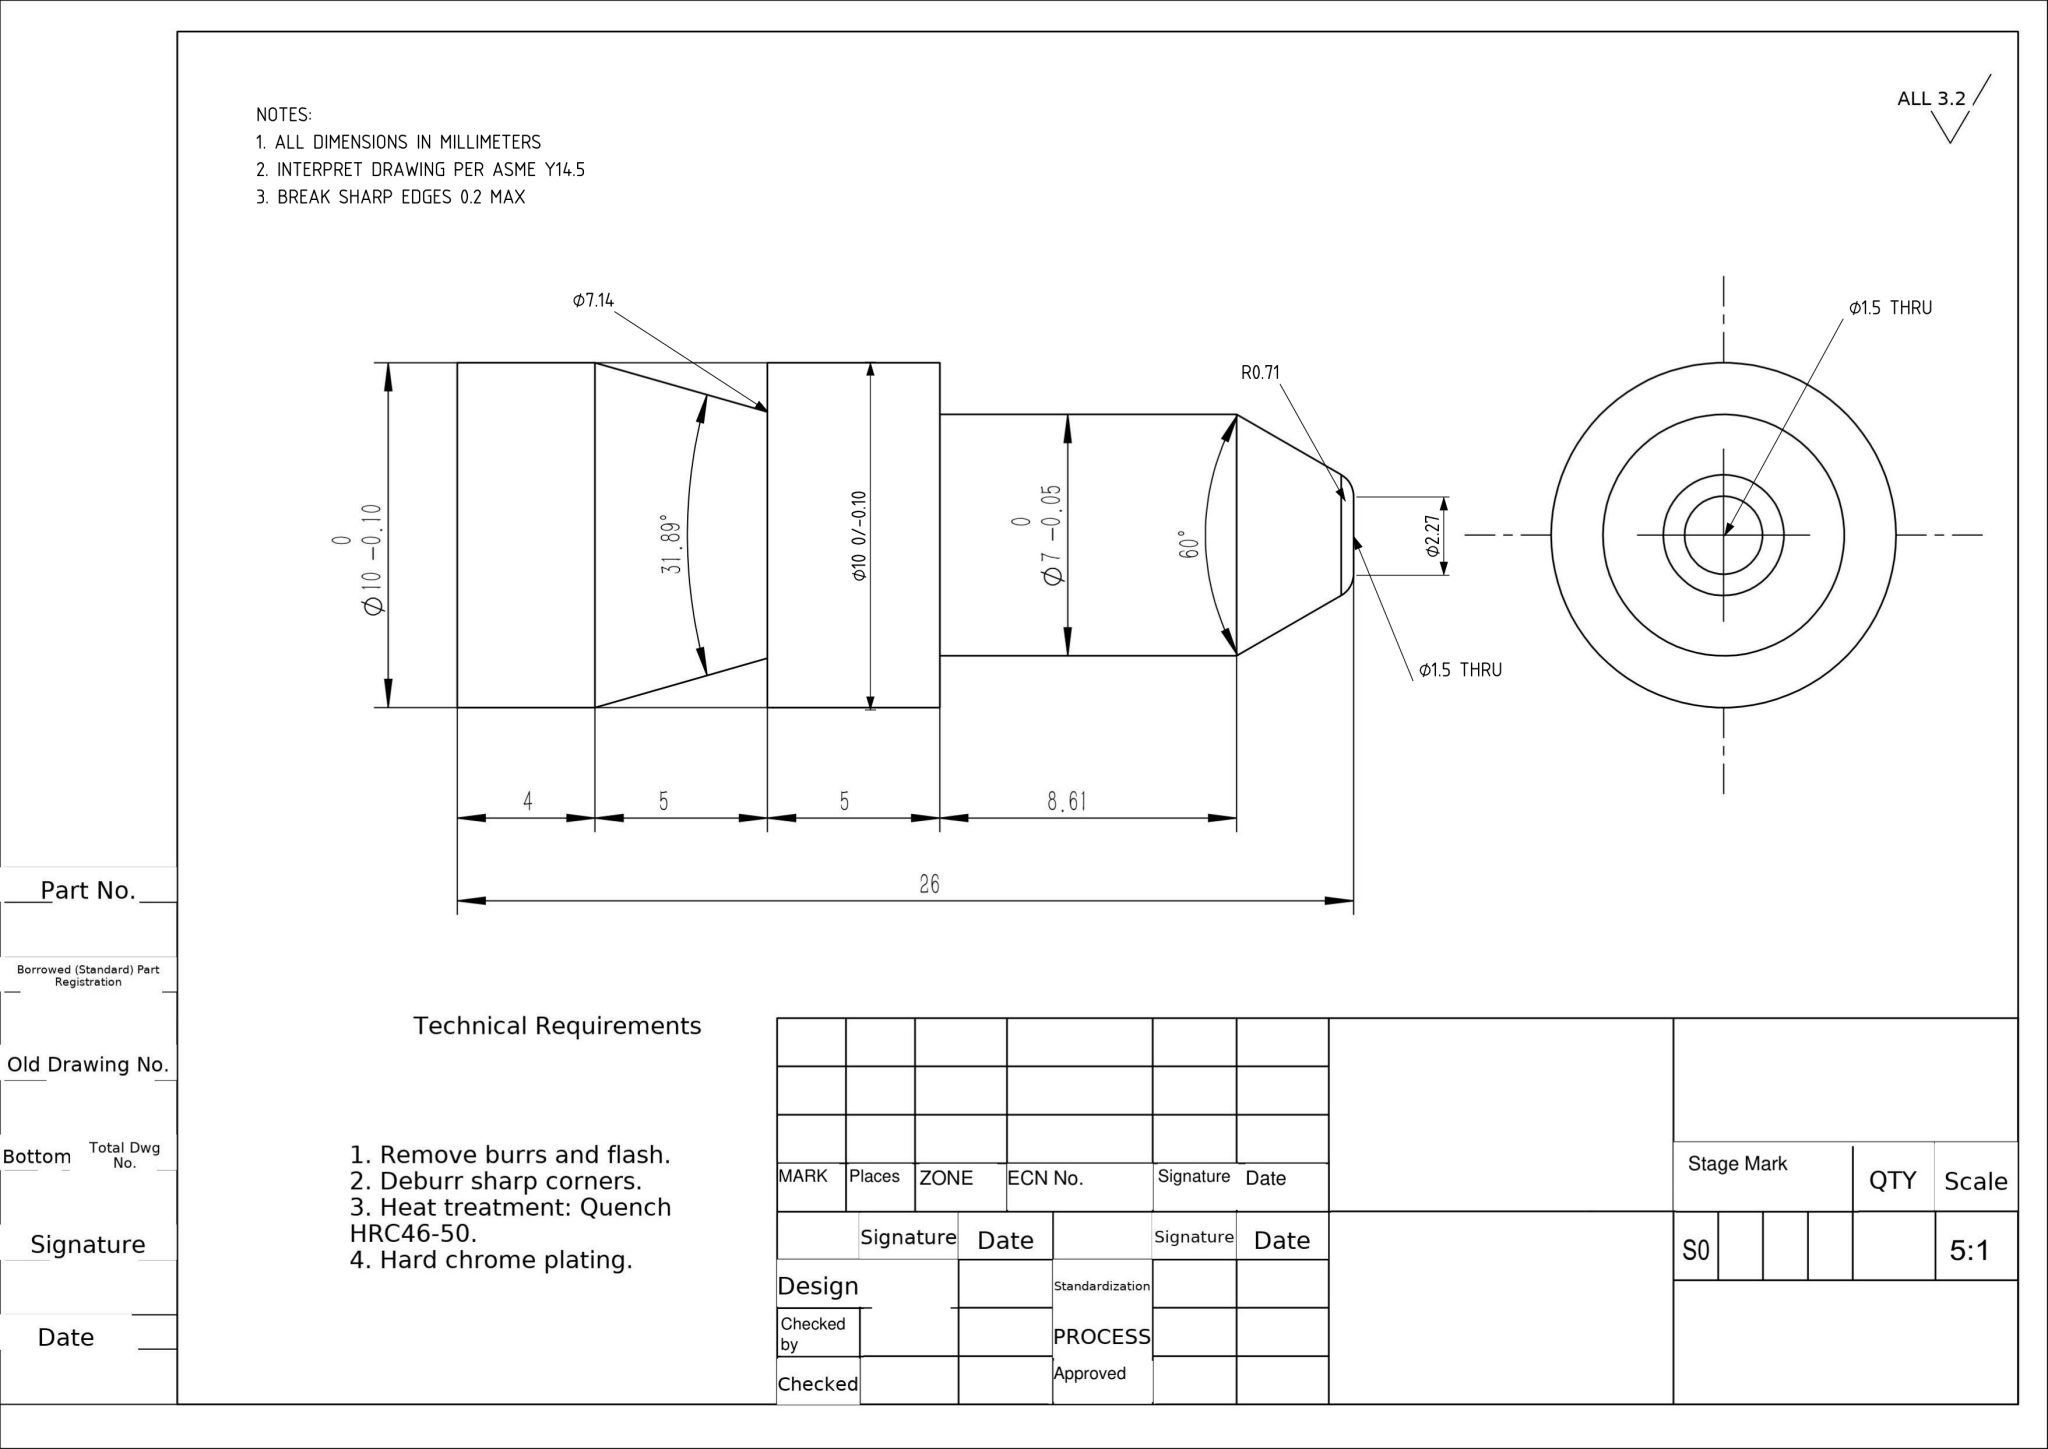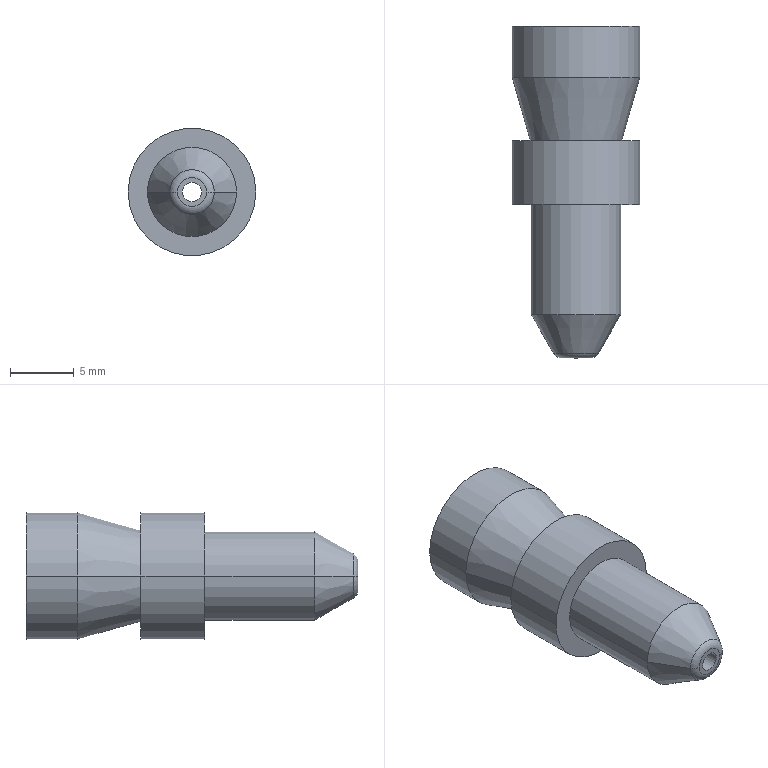Part | NX | mm | 1 solid | 18 faces | box 10 x 26 x 10 mm | volume 1354 mm3 | cylinder 8 | cone 4 | plane 4 | torus 2 | commonest cylinder face diameters 10 x4 1.5 x2 7 x2
STEP:
#1=COLOUR_RGB('',0.7922,0.8196,0.9333);
#2=FILL_AREA_STYLE_COLOUR('',#1);
#3=FILL_AREA_STYLE('',(#2));
#4=SURFACE_STYLE_FILL_AREA(#3);
#5=SURFACE_SIDE_STYLE('',(#4));
#6=SURFACE_STYLE_USAGE(.BOTH.,#5);
#7=PRESENTATION_STYLE_ASSIGNMENT((#6));
#8=CARTESIAN_POINT('',(1.464,7.397,0.));
#9=VERTEX_POINT('',#8);
#10=CARTESIAN_POINT('',(-0.03571,7.397,0.));
#11=VERTEX_POINT('',#10);
#12=CARTESIAN_POINT('',(0.7143,7.397,0.));
#13=DIRECTION('',(-0.,1.,0.));
#14=DIRECTION('',(-1.,0.,0.));
#15=AXIS2_PLACEMENT_3D('',#12,#13,#14);
#16=CIRCLE('',#15,0.75);
#17=EDGE_CURVE('',#9,#11,#16,.T.);
#18=ORIENTED_EDGE('',*,*,#17,.F.);
#19=CARTESIAN_POINT('',(1.464,33.397,0.));
#20=VERTEX_POINT('',#19);
#21=CARTESIAN_POINT('',(1.464,7.397,0.));
#22=DIRECTION('',(-0.,1.,0.));
#23=VECTOR('',#22,1000.);
#24=LINE('',#21,#23);
#25=EDGE_CURVE('',#9,#20,#24,.T.);
#26=ORIENTED_EDGE('',*,*,#25,.T.);
#27=CARTESIAN_POINT('',(-0.03571,33.397,0.));
#28=VERTEX_POINT('',#27);
#29=CARTESIAN_POINT('',(0.7143,33.397,0.));
#30=DIRECTION('',(-0.,1.,0.));
#31=DIRECTION('',(-1.,0.,0.));
#32=AXIS2_PLACEMENT_3D('',#29,#30,#31);
#33=CIRCLE('',#32,0.75);
#34=EDGE_CURVE('',#20,#28,#33,.T.);
#35=ORIENTED_EDGE('',*,*,#34,.T.);
#36=CARTESIAN_POINT('',(-0.03571,7.397,0.));
#37=DIRECTION('',(-0.,1.,0.));
#38=VECTOR('',#37,1000.);
#39=LINE('',#36,#38);
#40=EDGE_CURVE('',#11,#28,#39,.T.);
#41=ORIENTED_EDGE('',*,*,#40,.F.);
#42=EDGE_LOOP('',(#18,#26,#35,#41));
#43=FACE_OUTER_BOUND('',#42,.T.);
#44=CARTESIAN_POINT('',(0.7143,7.397,0.));
#45=DIRECTION('',(-0.,1.,0.));
#46=DIRECTION('',(-1.,0.,0.));
#47=AXIS2_PLACEMENT_3D('',#44,#45,#46);
#48=CYLINDRICAL_SURFACE('',#47,0.75);
#49=ADVANCED_FACE('',(#43),#48,.F.);
#50=CARTESIAN_POINT('',(2.464,7.755,0.));
#51=VERTEX_POINT('',#50);
#52=CARTESIAN_POINT('',(4.214,10.786,0.));
#53=VERTEX_POINT('',#52);
#54=CARTESIAN_POINT('',(4.214,10.786,0.));
#55=DIRECTION('',(0.5,0.866,0.));
#56=VECTOR('',#55,1000.);
#57=LINE('',#54,#56);
#58=EDGE_CURVE('',#51,#53,#57,.T.);
#59=ORIENTED_EDGE('',*,*,#58,.F.);
#60=CARTESIAN_POINT('',(-1.036,7.755,0.));
#61=VERTEX_POINT('',#60);
#62=CARTESIAN_POINT('',(0.7143,7.755,0.));
#63=DIRECTION('',(0.,1.,0.));
#64=DIRECTION('',(-1.,0.,0.));
#65=AXIS2_PLACEMENT_3D('',#62,#63,#64);
#66=CIRCLE('',#65,1.75);
#67=EDGE_CURVE('',#51,#61,#66,.T.);
#68=ORIENTED_EDGE('',*,*,#67,.T.);
#69=CARTESIAN_POINT('',(-2.786,10.786,0.));
#70=VERTEX_POINT('',#69);
#71=CARTESIAN_POINT('',(-2.786,10.786,0.));
#72=DIRECTION('',(-0.5,0.866,0.));
#73=VECTOR('',#72,1000.);
#74=LINE('',#71,#73);
#75=EDGE_CURVE('',#61,#70,#74,.T.);
#76=ORIENTED_EDGE('',*,*,#75,.T.);
#77=CARTESIAN_POINT('',(0.7143,10.786,0.));
#78=DIRECTION('',(0.,1.,0.));
#79=DIRECTION('',(-1.,0.,0.));
#80=AXIS2_PLACEMENT_3D('',#77,#78,#79);
#81=CIRCLE('',#80,3.5);
#82=EDGE_CURVE('',#53,#70,#81,.T.);
#83=ORIENTED_EDGE('',*,*,#82,.F.);
#84=EDGE_LOOP('',(#59,#68,#76,#83));
#85=FACE_OUTER_BOUND('',#84,.T.);
#86=CARTESIAN_POINT('',(0.7143,10.786,0.));
#87=DIRECTION('',(0.,1.,0.));
#88=DIRECTION('',(-1.,0.,0.));
#89=AXIS2_PLACEMENT_3D('',#86,#87,#88);
#90=CONICAL_SURFACE('',#89,3.5,0.5236);
#91=ADVANCED_FACE('',(#85),#90,.T.);
#92=CARTESIAN_POINT('',(4.214,19.397,0.));
#93=VERTEX_POINT('',#92);
#94=CARTESIAN_POINT('',(4.214,7.397,0.));
#95=DIRECTION('',(-0.,1.,0.));
#96=VECTOR('',#95,1000.);
#97=LINE('',#94,#96);
#98=EDGE_CURVE('',#53,#93,#97,.T.);
#99=ORIENTED_EDGE('',*,*,#98,.F.);
#100=ORIENTED_EDGE('',*,*,#82,.T.);
#101=CARTESIAN_POINT('',(-2.786,19.397,0.));
#102=VERTEX_POINT('',#101);
#103=CARTESIAN_POINT('',(-2.786,7.397,0.));
#104=DIRECTION('',(-0.,1.,0.));
#105=VECTOR('',#104,1000.);
#106=LINE('',#103,#105);
#107=EDGE_CURVE('',#70,#102,#106,.T.);
#108=ORIENTED_EDGE('',*,*,#107,.T.);
#109=CARTESIAN_POINT('',(0.7143,19.397,0.));
#110=DIRECTION('',(0.,1.,0.));
#111=DIRECTION('',(-1.,0.,0.));
#112=AXIS2_PLACEMENT_3D('',#109,#110,#111);
#113=CIRCLE('',#112,3.5);
#114=EDGE_CURVE('',#93,#102,#113,.T.);
#115=ORIENTED_EDGE('',*,*,#114,.F.);
#116=EDGE_LOOP('',(#99,#100,#108,#115));
#117=FACE_OUTER_BOUND('',#116,.T.);
#118=CARTESIAN_POINT('',(0.7143,7.397,0.));
#119=DIRECTION('',(0.,1.,0.));
#120=DIRECTION('',(-1.,0.,0.));
#121=AXIS2_PLACEMENT_3D('',#118,#119,#120);
#122=CYLINDRICAL_SURFACE('',#121,3.5);
#123=ADVANCED_FACE('',(#117),#122,.T.);
#124=CARTESIAN_POINT('',(0.7143,19.397,0.));
#125=DIRECTION('',(0.,1.,0.));
#126=DIRECTION('',(-1.,0.,0.));
#127=AXIS2_PLACEMENT_3D('',#124,#125,#126);
#128=CIRCLE('',#127,3.5);
#129=EDGE_CURVE('',#102,#93,#128,.T.);
#130=ORIENTED_EDGE('',*,*,#129,.T.);
#131=ORIENTED_EDGE('',*,*,#114,.T.);
#132=EDGE_LOOP('',(#130,#131));
#133=FACE_BOUND('',#132,.T.);
#134=CARTESIAN_POINT('',(-4.286,19.397,0.));
#135=VERTEX_POINT('',#134);
#136=CARTESIAN_POINT('',(5.714,19.397,0.));
#137=VERTEX_POINT('',#136);
#138=CARTESIAN_POINT('',(0.7143,19.397,0.));
#139=DIRECTION('',(0.,1.,0.));
#140=DIRECTION('',(-1.,0.,0.));
#141=AXIS2_PLACEMENT_3D('',#138,#139,#140);
#142=CIRCLE('',#141,5.);
#143=EDGE_CURVE('',#135,#137,#142,.T.);
#144=ORIENTED_EDGE('',*,*,#143,.F.);
#145=CARTESIAN_POINT('',(0.7143,19.397,0.));
#146=DIRECTION('',(0.,1.,0.));
#147=DIRECTION('',(-1.,0.,0.));
#148=AXIS2_PLACEMENT_3D('',#145,#146,#147);
#149=CIRCLE('',#148,5.);
#150=EDGE_CURVE('',#137,#135,#149,.T.);
#151=ORIENTED_EDGE('',*,*,#150,.F.);
#152=EDGE_LOOP('',(#144,#151));
#153=FACE_OUTER_BOUND('',#152,.T.);
#154=CARTESIAN_POINT('',(5.714,19.397,0.));
#155=DIRECTION('',(0.,-1.,0.));
#156=DIRECTION('',(0.,0.,-1.));
#157=AXIS2_PLACEMENT_3D('',#154,#155,#156);
#158=PLANE('',#157);
#159=ADVANCED_FACE('',(#133,#153),#158,.T.);
#160=CARTESIAN_POINT('',(5.714,24.397,0.));
#161=VERTEX_POINT('',#160);
#162=CARTESIAN_POINT('',(5.714,7.397,0.));
#163=DIRECTION('',(-0.,1.,0.));
#164=VECTOR('',#163,1000.);
#165=LINE('',#162,#164);
#166=EDGE_CURVE('',#137,#161,#165,.T.);
#167=ORIENTED_EDGE('',*,*,#166,.F.);
#168=ORIENTED_EDGE('',*,*,#150,.T.);
#169=CARTESIAN_POINT('',(-4.286,24.397,0.));
#170=VERTEX_POINT('',#169);
#171=CARTESIAN_POINT('',(-4.286,7.397,0.));
#172=DIRECTION('',(-0.,1.,0.));
#173=VECTOR('',#172,1000.);
#174=LINE('',#171,#173);
#175=EDGE_CURVE('',#135,#170,#174,.T.);
#176=ORIENTED_EDGE('',*,*,#175,.T.);
#177=CARTESIAN_POINT('',(0.7143,24.397,0.));
#178=DIRECTION('',(0.,1.,0.));
#179=DIRECTION('',(-1.,0.,0.));
#180=AXIS2_PLACEMENT_3D('',#177,#178,#179);
#181=CIRCLE('',#180,5.);
#182=EDGE_CURVE('',#161,#170,#181,.T.);
#183=ORIENTED_EDGE('',*,*,#182,.F.);
#184=EDGE_LOOP('',(#167,#168,#176,#183));
#185=FACE_OUTER_BOUND('',#184,.T.);
#186=CARTESIAN_POINT('',(0.7143,7.397,0.));
#187=DIRECTION('',(0.,1.,0.));
#188=DIRECTION('',(-1.,0.,0.));
#189=AXIS2_PLACEMENT_3D('',#186,#187,#188);
#190=CYLINDRICAL_SURFACE('',#189,5.);
#191=ADVANCED_FACE('',(#185),#190,.T.);
#192=CARTESIAN_POINT('',(-2.857,24.397,0.));
#193=VERTEX_POINT('',#192);
#194=CARTESIAN_POINT('',(4.286,24.397,0.));
#195=VERTEX_POINT('',#194);
#196=CARTESIAN_POINT('',(0.7143,24.397,0.));
#197=DIRECTION('',(0.,1.,0.));
#198=DIRECTION('',(-1.,0.,0.));
#199=AXIS2_PLACEMENT_3D('',#196,#197,#198);
#200=CIRCLE('',#199,3.571);
#201=EDGE_CURVE('',#193,#195,#200,.T.);
#202=ORIENTED_EDGE('',*,*,#201,.F.);
#203=CARTESIAN_POINT('',(0.7143,24.397,0.));
#204=DIRECTION('',(0.,1.,0.));
#205=DIRECTION('',(-1.,0.,0.));
#206=AXIS2_PLACEMENT_3D('',#203,#204,#205);
#207=CIRCLE('',#206,3.571);
#208=EDGE_CURVE('',#195,#193,#207,.T.);
#209=ORIENTED_EDGE('',*,*,#208,.F.);
#210=EDGE_LOOP('',(#202,#209));
#211=FACE_BOUND('',#210,.T.);
#212=CARTESIAN_POINT('',(0.7143,24.397,0.));
#213=DIRECTION('',(0.,1.,0.));
#214=DIRECTION('',(-1.,0.,0.));
#215=AXIS2_PLACEMENT_3D('',#212,#213,#214);
#216=CIRCLE('',#215,5.);
#217=EDGE_CURVE('',#170,#161,#216,.T.);
#218=ORIENTED_EDGE('',*,*,#217,.T.);
#219=ORIENTED_EDGE('',*,*,#182,.T.);
#220=EDGE_LOOP('',(#218,#219));
#221=FACE_OUTER_BOUND('',#220,.T.);
#222=CARTESIAN_POINT('',(4.286,24.397,0.));
#223=DIRECTION('',(-0.,1.,0.));
#224=DIRECTION('',(1.,0.,0.));
#225=AXIS2_PLACEMENT_3D('',#222,#223,#224);
#226=PLANE('',#225);
#227=ADVANCED_FACE('',(#211,#221),#226,.T.);
#228=CARTESIAN_POINT('',(5.714,29.397,0.));
#229=VERTEX_POINT('',#228);
#230=CARTESIAN_POINT('',(5.714,29.397,0.));
#231=DIRECTION('',(0.2747,0.9615,0.));
#232=VECTOR('',#231,1000.);
#233=LINE('',#230,#232);
#234=EDGE_CURVE('',#195,#229,#233,.T.);
#235=ORIENTED_EDGE('',*,*,#234,.F.);
#236=ORIENTED_EDGE('',*,*,#208,.T.);
#237=CARTESIAN_POINT('',(-4.286,29.397,0.));
#238=VERTEX_POINT('',#237);
#239=CARTESIAN_POINT('',(-4.286,29.397,0.));
#240=DIRECTION('',(-0.2747,0.9615,0.));
#241=VECTOR('',#240,1000.);
#242=LINE('',#239,#241);
#243=EDGE_CURVE('',#193,#238,#242,.T.);
#244=ORIENTED_EDGE('',*,*,#243,.T.);
#245=CARTESIAN_POINT('',(0.7143,29.397,0.));
#246=DIRECTION('',(0.,1.,0.));
#247=DIRECTION('',(-1.,0.,0.));
#248=AXIS2_PLACEMENT_3D('',#245,#246,#247);
#249=CIRCLE('',#248,5.);
#250=EDGE_CURVE('',#229,#238,#249,.T.);
#251=ORIENTED_EDGE('',*,*,#250,.F.);
#252=EDGE_LOOP('',(#235,#236,#244,#251));
#253=FACE_OUTER_BOUND('',#252,.T.);
#254=CARTESIAN_POINT('',(0.7143,29.397,0.));
#255=DIRECTION('',(0.,1.,0.));
#256=DIRECTION('',(-1.,0.,0.));
#257=AXIS2_PLACEMENT_3D('',#254,#255,#256);
#258=CONICAL_SURFACE('',#257,5.,0.2783);
#259=ADVANCED_FACE('',(#253),#258,.T.);
#260=CARTESIAN_POINT('',(5.714,33.397,0.));
#261=VERTEX_POINT('',#260);
#262=CARTESIAN_POINT('',(5.714,7.397,0.));
#263=DIRECTION('',(-0.,1.,0.));
#264=VECTOR('',#263,1000.);
#265=LINE('',#262,#264);
#266=EDGE_CURVE('',#229,#261,#265,.T.);
#267=ORIENTED_EDGE('',*,*,#266,.F.);
#268=ORIENTED_EDGE('',*,*,#250,.T.);
#269=CARTESIAN_POINT('',(-4.286,33.397,0.));
#270=VERTEX_POINT('',#269);
#271=CARTESIAN_POINT('',(-4.286,7.397,0.));
#272=DIRECTION('',(-0.,1.,0.));
#273=VECTOR('',#272,1000.);
#274=LINE('',#271,#273);
#275=EDGE_CURVE('',#238,#270,#274,.T.);
#276=ORIENTED_EDGE('',*,*,#275,.T.);
#277=CARTESIAN_POINT('',(0.7143,33.397,0.));
#278=DIRECTION('',(0.,1.,0.));
#279=DIRECTION('',(-1.,0.,0.));
#280=AXIS2_PLACEMENT_3D('',#277,#278,#279);
#281=CIRCLE('',#280,5.);
#282=EDGE_CURVE('',#261,#270,#281,.T.);
#283=ORIENTED_EDGE('',*,*,#282,.F.);
#284=EDGE_LOOP('',(#267,#268,#276,#283));
#285=FACE_OUTER_BOUND('',#284,.T.);
#286=CARTESIAN_POINT('',(0.7143,7.397,0.));
#287=DIRECTION('',(0.,1.,0.));
#288=DIRECTION('',(-1.,0.,0.));
#289=AXIS2_PLACEMENT_3D('',#286,#287,#288);
#290=CYLINDRICAL_SURFACE('',#289,5.);
#291=ADVANCED_FACE('',(#285),#290,.T.);
#292=CARTESIAN_POINT('',(0.7143,33.397,0.));
#293=DIRECTION('',(-0.,1.,0.));
#294=DIRECTION('',(-1.,0.,0.));
#295=AXIS2_PLACEMENT_3D('',#292,#293,#294);
#296=CIRCLE('',#295,0.75);
#297=EDGE_CURVE('',#28,#20,#296,.T.);
#298=ORIENTED_EDGE('',*,*,#297,.F.);
#299=ORIENTED_EDGE('',*,*,#34,.F.);
#300=EDGE_LOOP('',(#298,#299));
#301=FACE_BOUND('',#300,.T.);
#302=CARTESIAN_POINT('',(0.7143,33.397,0.));
#303=DIRECTION('',(0.,1.,0.));
#304=DIRECTION('',(-1.,0.,0.));
#305=AXIS2_PLACEMENT_3D('',#302,#303,#304);
#306=CIRCLE('',#305,5.);
#307=EDGE_CURVE('',#270,#261,#306,.T.);
#308=ORIENTED_EDGE('',*,*,#307,.T.);
#309=ORIENTED_EDGE('',*,*,#282,.T.);
#310=EDGE_LOOP('',(#308,#309));
#311=FACE_OUTER_BOUND('',#310,.T.);
#312=CARTESIAN_POINT('',(0.7143,33.397,0.));
#313=DIRECTION('',(-0.,1.,0.));
#314=DIRECTION('',(1.,0.,0.));
#315=AXIS2_PLACEMENT_3D('',#312,#313,#314);
#316=PLANE('',#315);
#317=ADVANCED_FACE('',(#301,#311),#316,.T.);
#318=CARTESIAN_POINT('',(0.7143,7.397,0.));
#319=DIRECTION('',(-0.,1.,0.));
#320=DIRECTION('',(-1.,0.,0.));
#321=AXIS2_PLACEMENT_3D('',#318,#319,#320);
#322=CIRCLE('',#321,0.75);
#323=EDGE_CURVE('',#11,#9,#322,.T.);
#324=ORIENTED_EDGE('',*,*,#323,.T.);
#325=ORIENTED_EDGE('',*,*,#17,.T.);
#326=EDGE_LOOP('',(#324,#325));
#327=FACE_BOUND('',#326,.T.);
#328=CARTESIAN_POINT('',(-0.4171,7.397,0.));
#329=VERTEX_POINT('',#328);
#330=CARTESIAN_POINT('',(1.846,7.397,0.));
#331=VERTEX_POINT('',#330);
#332=CARTESIAN_POINT('',(0.7143,7.397,0.));
#333=DIRECTION('',(0.,1.,0.));
#334=DIRECTION('',(-1.,0.,0.));
#335=AXIS2_PLACEMENT_3D('',#332,#333,#334);
#336=CIRCLE('',#335,1.131);
#337=EDGE_CURVE('',#329,#331,#336,.T.);
#338=ORIENTED_EDGE('',*,*,#337,.F.);
#339=CARTESIAN_POINT('',(0.7143,7.397,0.));
#340=DIRECTION('',(0.,1.,0.));
#341=DIRECTION('',(-1.,0.,0.));
#342=AXIS2_PLACEMENT_3D('',#339,#340,#341);
#343=CIRCLE('',#342,1.131);
#344=EDGE_CURVE('',#331,#329,#343,.T.);
#345=ORIENTED_EDGE('',*,*,#344,.F.);
#346=EDGE_LOOP('',(#338,#345));
#347=FACE_OUTER_BOUND('',#346,.T.);
#348=CARTESIAN_POINT('',(1.846,7.397,0.));
#349=DIRECTION('',(0.,-1.,0.));
#350=DIRECTION('',(0.,0.,-1.));
#351=AXIS2_PLACEMENT_3D('',#348,#349,#350);
#352=PLANE('',#351);
#353=ADVANCED_FACE('',(#327,#347),#352,.T.);
#354=CARTESIAN_POINT('',(1.846,8.112,0.));
#355=DIRECTION('',(-0.,-0.,1.));
#356=DIRECTION('',(1.,0.,0.));
#357=AXIS2_PLACEMENT_3D('',#354,#355,#356);
#358=CIRCLE('',#357,0.7143);
#359=EDGE_CURVE('',#331,#51,#358,.T.);
#360=ORIENTED_EDGE('',*,*,#359,.F.);
#361=ORIENTED_EDGE('',*,*,#344,.T.);
#362=CARTESIAN_POINT('',(-0.4171,8.112,0.));
#363=DIRECTION('',(0.,0.,-1.));
#364=DIRECTION('',(-1.,0.,0.));
#365=AXIS2_PLACEMENT_3D('',#362,#363,#364);
#366=CIRCLE('',#365,0.7143);
#367=EDGE_CURVE('',#329,#61,#366,.T.);
#368=ORIENTED_EDGE('',*,*,#367,.T.);
#369=ORIENTED_EDGE('',*,*,#67,.F.);
#370=EDGE_LOOP('',(#360,#361,#368,#369));
#371=FACE_OUTER_BOUND('',#370,.T.);
#372=CARTESIAN_POINT('',(0.7143,8.112,0.));
#373=DIRECTION('',(-0.,1.,0.));
#374=DIRECTION('',(-1.,-0.,0.));
#375=AXIS2_PLACEMENT_3D('',#372,#373,#374);
#376=TOROIDAL_SURFACE('',#375,1.131,0.7143);
#377=ADVANCED_FACE('',(#371),#376,.T.);
#378=ORIENTED_EDGE('',*,*,#337,.T.);
#379=ORIENTED_EDGE('',*,*,#359,.T.);
#380=CARTESIAN_POINT('',(0.7143,7.755,0.));
#381=DIRECTION('',(0.,1.,0.));
#382=DIRECTION('',(-1.,0.,0.));
#383=AXIS2_PLACEMENT_3D('',#380,#381,#382);
#384=CIRCLE('',#383,1.75);
#385=EDGE_CURVE('',#61,#51,#384,.T.);
#386=ORIENTED_EDGE('',*,*,#385,.F.);
#387=ORIENTED_EDGE('',*,*,#367,.F.);
#388=EDGE_LOOP('',(#378,#379,#386,#387));
#389=FACE_OUTER_BOUND('',#388,.T.);
#390=CARTESIAN_POINT('',(0.7143,8.112,0.));
#391=DIRECTION('',(-0.,1.,0.));
#392=DIRECTION('',(-1.,-0.,0.));
#393=AXIS2_PLACEMENT_3D('',#390,#391,#392);
#394=TOROIDAL_SURFACE('',#393,1.131,0.7143);
#395=ADVANCED_FACE('',(#389),#394,.T.);
#396=CARTESIAN_POINT('',(0.7143,29.397,0.));
#397=DIRECTION('',(0.,1.,0.));
#398=DIRECTION('',(-1.,0.,0.));
#399=AXIS2_PLACEMENT_3D('',#396,#397,#398);
#400=CIRCLE('',#399,5.);
#401=EDGE_CURVE('',#238,#229,#400,.T.);
#402=ORIENTED_EDGE('',*,*,#401,.T.);
#403=ORIENTED_EDGE('',*,*,#266,.T.);
#404=ORIENTED_EDGE('',*,*,#307,.F.);
#405=ORIENTED_EDGE('',*,*,#275,.F.);
#406=EDGE_LOOP('',(#402,#403,#404,#405));
#407=FACE_OUTER_BOUND('',#406,.T.);
#408=CARTESIAN_POINT('',(0.7143,7.397,0.));
#409=DIRECTION('',(0.,1.,0.));
#410=DIRECTION('',(-1.,0.,0.));
#411=AXIS2_PLACEMENT_3D('',#408,#409,#410);
#412=CYLINDRICAL_SURFACE('',#411,5.);
#413=ADVANCED_FACE('',(#407),#412,.T.);
#414=ORIENTED_EDGE('',*,*,#201,.T.);
#415=ORIENTED_EDGE('',*,*,#234,.T.);
#416=ORIENTED_EDGE('',*,*,#401,.F.);
#417=ORIENTED_EDGE('',*,*,#243,.F.);
#418=EDGE_LOOP('',(#414,#415,#416,#417));
#419=FACE_OUTER_BOUND('',#418,.T.);
#420=CARTESIAN_POINT('',(0.7143,29.397,0.));
#421=DIRECTION('',(0.,1.,0.));
#422=DIRECTION('',(-1.,0.,0.));
#423=AXIS2_PLACEMENT_3D('',#420,#421,#422);
#424=CONICAL_SURFACE('',#423,5.,0.2783);
#425=ADVANCED_FACE('',(#419),#424,.T.);
#426=ORIENTED_EDGE('',*,*,#143,.T.);
#427=ORIENTED_EDGE('',*,*,#166,.T.);
#428=ORIENTED_EDGE('',*,*,#217,.F.);
#429=ORIENTED_EDGE('',*,*,#175,.F.);
#430=EDGE_LOOP('',(#426,#427,#428,#429));
#431=FACE_OUTER_BOUND('',#430,.T.);
#432=CARTESIAN_POINT('',(0.7143,7.397,0.));
#433=DIRECTION('',(0.,1.,0.));
#434=DIRECTION('',(-1.,0.,0.));
#435=AXIS2_PLACEMENT_3D('',#432,#433,#434);
#436=CYLINDRICAL_SURFACE('',#435,5.);
#437=ADVANCED_FACE('',(#431),#436,.T.);
#438=CARTESIAN_POINT('',(0.7143,10.786,0.));
#439=DIRECTION('',(0.,1.,0.));
#440=DIRECTION('',(-1.,0.,0.));
#441=AXIS2_PLACEMENT_3D('',#438,#439,#440);
#442=CIRCLE('',#441,3.5);
#443=EDGE_CURVE('',#70,#53,#442,.T.);
#444=ORIENTED_EDGE('',*,*,#443,.T.);
#445=ORIENTED_EDGE('',*,*,#98,.T.);
#446=ORIENTED_EDGE('',*,*,#129,.F.);
#447=ORIENTED_EDGE('',*,*,#107,.F.);
#448=EDGE_LOOP('',(#444,#445,#446,#447));
#449=FACE_OUTER_BOUND('',#448,.T.);
#450=CARTESIAN_POINT('',(0.7143,7.397,0.));
#451=DIRECTION('',(0.,1.,0.));
#452=DIRECTION('',(-1.,0.,0.));
#453=AXIS2_PLACEMENT_3D('',#450,#451,#452);
#454=CYLINDRICAL_SURFACE('',#453,3.5);
#455=ADVANCED_FACE('',(#449),#454,.T.);
#456=ORIENTED_EDGE('',*,*,#385,.T.);
#457=ORIENTED_EDGE('',*,*,#58,.T.);
#458=ORIENTED_EDGE('',*,*,#443,.F.);
#459=ORIENTED_EDGE('',*,*,#75,.F.);
#460=EDGE_LOOP('',(#456,#457,#458,#459));
#461=FACE_OUTER_BOUND('',#460,.T.);
#462=CARTESIAN_POINT('',(0.7143,10.786,0.));
#463=DIRECTION('',(0.,1.,0.));
#464=DIRECTION('',(-1.,0.,0.));
#465=AXIS2_PLACEMENT_3D('',#462,#463,#464);
#466=CONICAL_SURFACE('',#465,3.5,0.5236);
#467=ADVANCED_FACE('',(#461),#466,.T.);
#468=ORIENTED_EDGE('',*,*,#25,.F.);
#469=ORIENTED_EDGE('',*,*,#323,.F.);
#470=ORIENTED_EDGE('',*,*,#40,.T.);
#471=ORIENTED_EDGE('',*,*,#297,.T.);
#472=EDGE_LOOP('',(#468,#469,#470,#471));
#473=FACE_OUTER_BOUND('',#472,.T.);
#474=CARTESIAN_POINT('',(0.7143,7.397,0.));
#475=DIRECTION('',(-0.,1.,0.));
#476=DIRECTION('',(-1.,0.,0.));
#477=AXIS2_PLACEMENT_3D('',#474,#475,#476);
#478=CYLINDRICAL_SURFACE('',#477,0.75);
#479=ADVANCED_FACE('',(#473),#478,.F.);
#480=CLOSED_SHELL('',(#49,#91,#123,#159,#191,#227,#259,#291,#317,#353,#377,#395,#413,#425,#437,#455,#467,#479));
#481=MANIFOLD_SOLID_BREP('',#480);
#482=STYLED_ITEM('',(#7),#481);
#483=(LENGTH_UNIT()NAMED_UNIT(*)SI_UNIT(.MILLI.,.METRE.));
#484=UNCERTAINTY_MEASURE_WITH_UNIT(LENGTH_MEASURE(0.00001),#483,'','');
#485=(NAMED_UNIT(*)PLANE_ANGLE_UNIT()SI_UNIT($,.RADIAN.));
#486=(NAMED_UNIT(*)SI_UNIT($,.STERADIAN.)SOLID_ANGLE_UNIT());
#487=(GEOMETRIC_REPRESENTATION_CONTEXT(3)GLOBAL_UNCERTAINTY_ASSIGNED_CONTEXT((#484))GLOBAL_UNIT_ASSIGNED_CONTEXT((#483,#485,#486))REPRESENTATION_CONTEXT('',''));
#488=MECHANICAL_DESIGN_GEOMETRIC_PRESENTATION_REPRESENTATION('',(#482),#487);
#489=PRESENTATION_LAYER_ASSIGNMENT('','',(#482));
#490=CARTESIAN_POINT('',(0.,0.,0.));
#491=DIRECTION('',(0.,0.,1.));
#492=DIRECTION('',(1.,0.,0.));
#493=AXIS2_PLACEMENT_3D('',#490,#491,#492);
#494=(LENGTH_UNIT()NAMED_UNIT(*)SI_UNIT(.MILLI.,.METRE.));
#495=UNCERTAINTY_MEASURE_WITH_UNIT(LENGTH_MEASURE(0.00001),#494,'','');
#496=(NAMED_UNIT(*)PLANE_ANGLE_UNIT()SI_UNIT($,.RADIAN.));
#497=(NAMED_UNIT(*)SI_UNIT($,.STERADIAN.)SOLID_ANGLE_UNIT());
#498=(GEOMETRIC_REPRESENTATION_CONTEXT(3)GLOBAL_UNCERTAINTY_ASSIGNED_CONTEXT((#495))GLOBAL_UNIT_ASSIGNED_CONTEXT((#494,#496,#497))REPRESENTATION_CONTEXT('',''));
#499=ADVANCED_BREP_SHAPE_REPRESENTATION('',(#481,#493),#498);